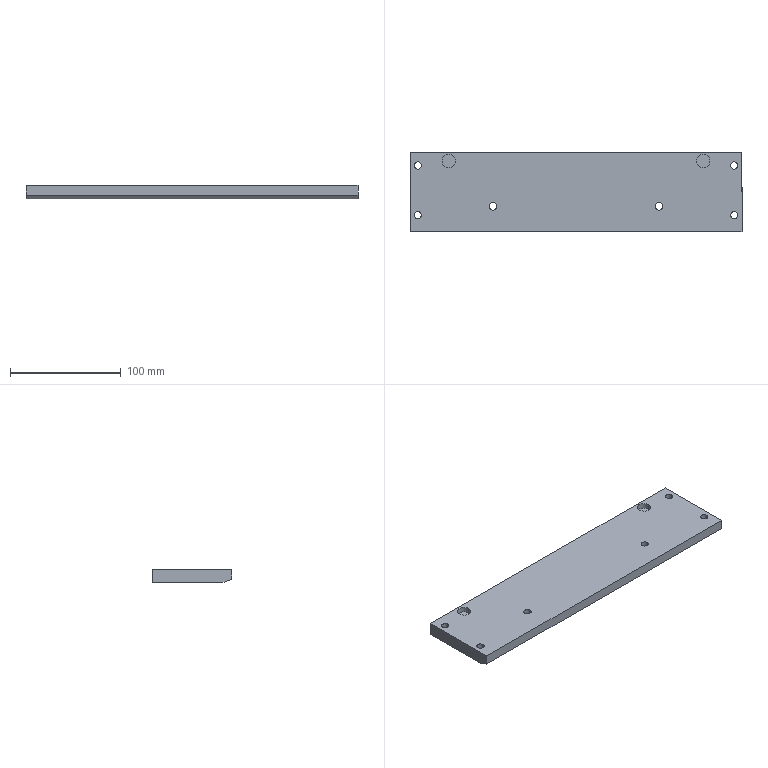Component | SolidWorks | OPW-05-006-1 | 1 solid | 43 faces | box 300 x 72 x 12 mm | volume 249816 mm3 | cylinder 28 | plane 15 | commonest cylinder face diameters 11 x12 6.6 x12 12 x4
build123d program:
from build123d import *

# Parameters (mm, degrees)
SKETCH1_W                                       = 300
SKETCH1_H                                       = 72
BOSS_EXTRUDE1_DEPTH                             = 6
M6_HEX_SOCKET_HEAD_CAP_SCREW_CBORE1_D           = 6.6
M6_HEX_SOCKET_HEAD_CAP_SCREW_CBORE1_CBORE_D     = 11
M6_HEX_SOCKET_HEAD_CAP_SCREW_CBORE1_CBORE_DEPTH = 6
SKETCH7_R                                       = 6
CUT_EXTRUDE2_DEPTH                              = 5
CHAMFER1_SIZE                                   = 3
CHAMFER1_SIZE2                                  = 8
M6_HEX_SOCKET_HEAD_CAP_SCREW_CBORE2_D           = 6.6
M6_HEX_SOCKET_HEAD_CAP_SCREW_CBORE2_CBORE_D     = 11
M6_HEX_SOCKET_HEAD_CAP_SCREW_CBORE2_CBORE_DEPTH = 6


with BuildPart() as part:
    # Sketch1 → Boss-Extrude1 (new, symmetric)
    with BuildSketch(Plane.XY):
        Rectangle(SKETCH1_W, SKETCH1_H)
    extrude(amount=BOSS_EXTRUDE1_DEPTH, both=True)

    # M6 Hex Socket Head Cap Screw CBORE1 (through all)
    with Locations(Plane.XY.offset(6)):
        with Locations((-143, 24), (-143, -21), (143, 24), (143, -21)):
            CounterBoreHole(M6_HEX_SOCKET_HEAD_CAP_SCREW_CBORE1_D / 2, M6_HEX_SOCKET_HEAD_CAP_SCREW_CBORE1_CBORE_D / 2, M6_HEX_SOCKET_HEAD_CAP_SCREW_CBORE1_CBORE_DEPTH)

    # Sketch7 → Cut-Extrude2 (cut)
    with BuildSketch(Plane(origin=(0, 0, -6), x_dir=(-1, 0, 0), z_dir=(0, 0, -1))):
        with Locations((115, 28)):
            Circle(SKETCH7_R)
        with Locations((-115, 28)):
            Circle(SKETCH7_R)
    extrude(amount=-CUT_EXTRUDE2_DEPTH, mode=Mode.SUBTRACT)

    # Chamfer1
    chamfer1_edges = [part.edges().sort_by_distance(p)[0] for p in [
        (0, -36, 6),
    ]]
    chamfer1_side = [part.faces().sort_by_distance(p)[0] for p in [
        (0, -36, 0),
    ]]
    chamfer(chamfer1_edges, length=CHAMFER1_SIZE, length2=CHAMFER1_SIZE2, reference=chamfer1_side[0])

    # M6 Hex Socket Head Cap Screw CBORE2 (through all)
    with Locations(Plane.XY.offset(6)):
        with Locations((-75, -13), (75, -13)):
            CounterBoreHole(M6_HEX_SOCKET_HEAD_CAP_SCREW_CBORE2_D / 2, M6_HEX_SOCKET_HEAD_CAP_SCREW_CBORE2_CBORE_D / 2, M6_HEX_SOCKET_HEAD_CAP_SCREW_CBORE2_CBORE_DEPTH)


solid = part.part

# Placed as in the assembly
solid = solid.moved(Location((-104.904, 162.999, -36), (-180, 0, 180)))